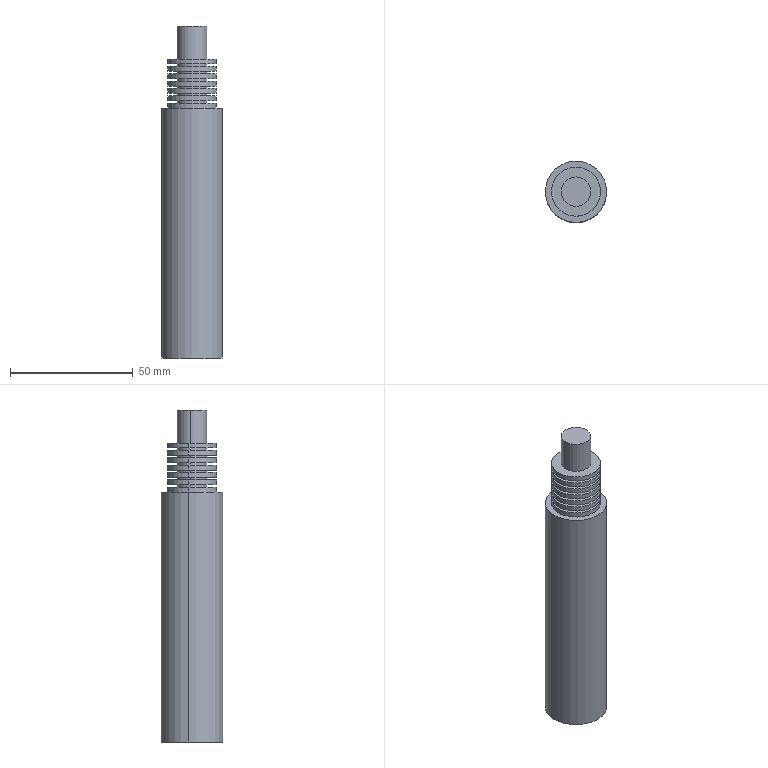Component | SolidWorks | Motor-2 | 1 solid | 46 faces | box 25 x 25 x 135.5 mm | volume 56673 mm3 | cylinder 30 | plane 16 | commonest cylinder face diameters 12 x14 20 x14 25 x2
build123d program:
from build123d import *

# Parameters (mm, degrees)
BOSS_EXTRUDE1_DEPTH      = 20
BOSS_EXTRUDE1_DEPTH_BACK = 11.5
SKETCH1_R                = 6
SKETCH2_R                = 10
BOSS_EXTRUDE2_DEPTH      = 2
LPATTERN1_COUNT          = 7
LPATTERN1_PITCH          = 3
SKETCH3_R                = 12.5
BOSS_EXTRUDE3_DEPTH      = 102


with BuildPart() as part:
    # Sketch1 → Boss-Extrude1 (new, two sides: drawn at the far end of the back side and taken through both)
    with BuildSketch(Plane.XY.offset(-BOSS_EXTRUDE1_DEPTH_BACK)):
        Circle(SKETCH1_R)
    extrude(amount=BOSS_EXTRUDE1_DEPTH + BOSS_EXTRUDE1_DEPTH_BACK)

    # Sketch2 → Boss-Extrude2 (add)
    with BuildSketch(Plane.XY.offset(20)):
        Circle(SKETCH2_R)
    boss_extrude2 = extrude(amount=BOSS_EXTRUDE2_DEPTH)

    # LPattern1: Boss-Extrude2 ×7
    with Locations(*[(0, 0, -i * LPATTERN1_PITCH) for i in range(1, LPATTERN1_COUNT)]):
        add(boss_extrude2)

    # Sketch3 → Boss-Extrude3 (add)
    with BuildSketch(Plane.XY.offset(22)):
        Circle(SKETCH3_R)
    extrude(amount=BOSS_EXTRUDE3_DEPTH)


solid = part.part

# Placed as in the assembly
solid = solid.moved(Location((-24.375, -67.172, 24.182), (180, 0, 0)))